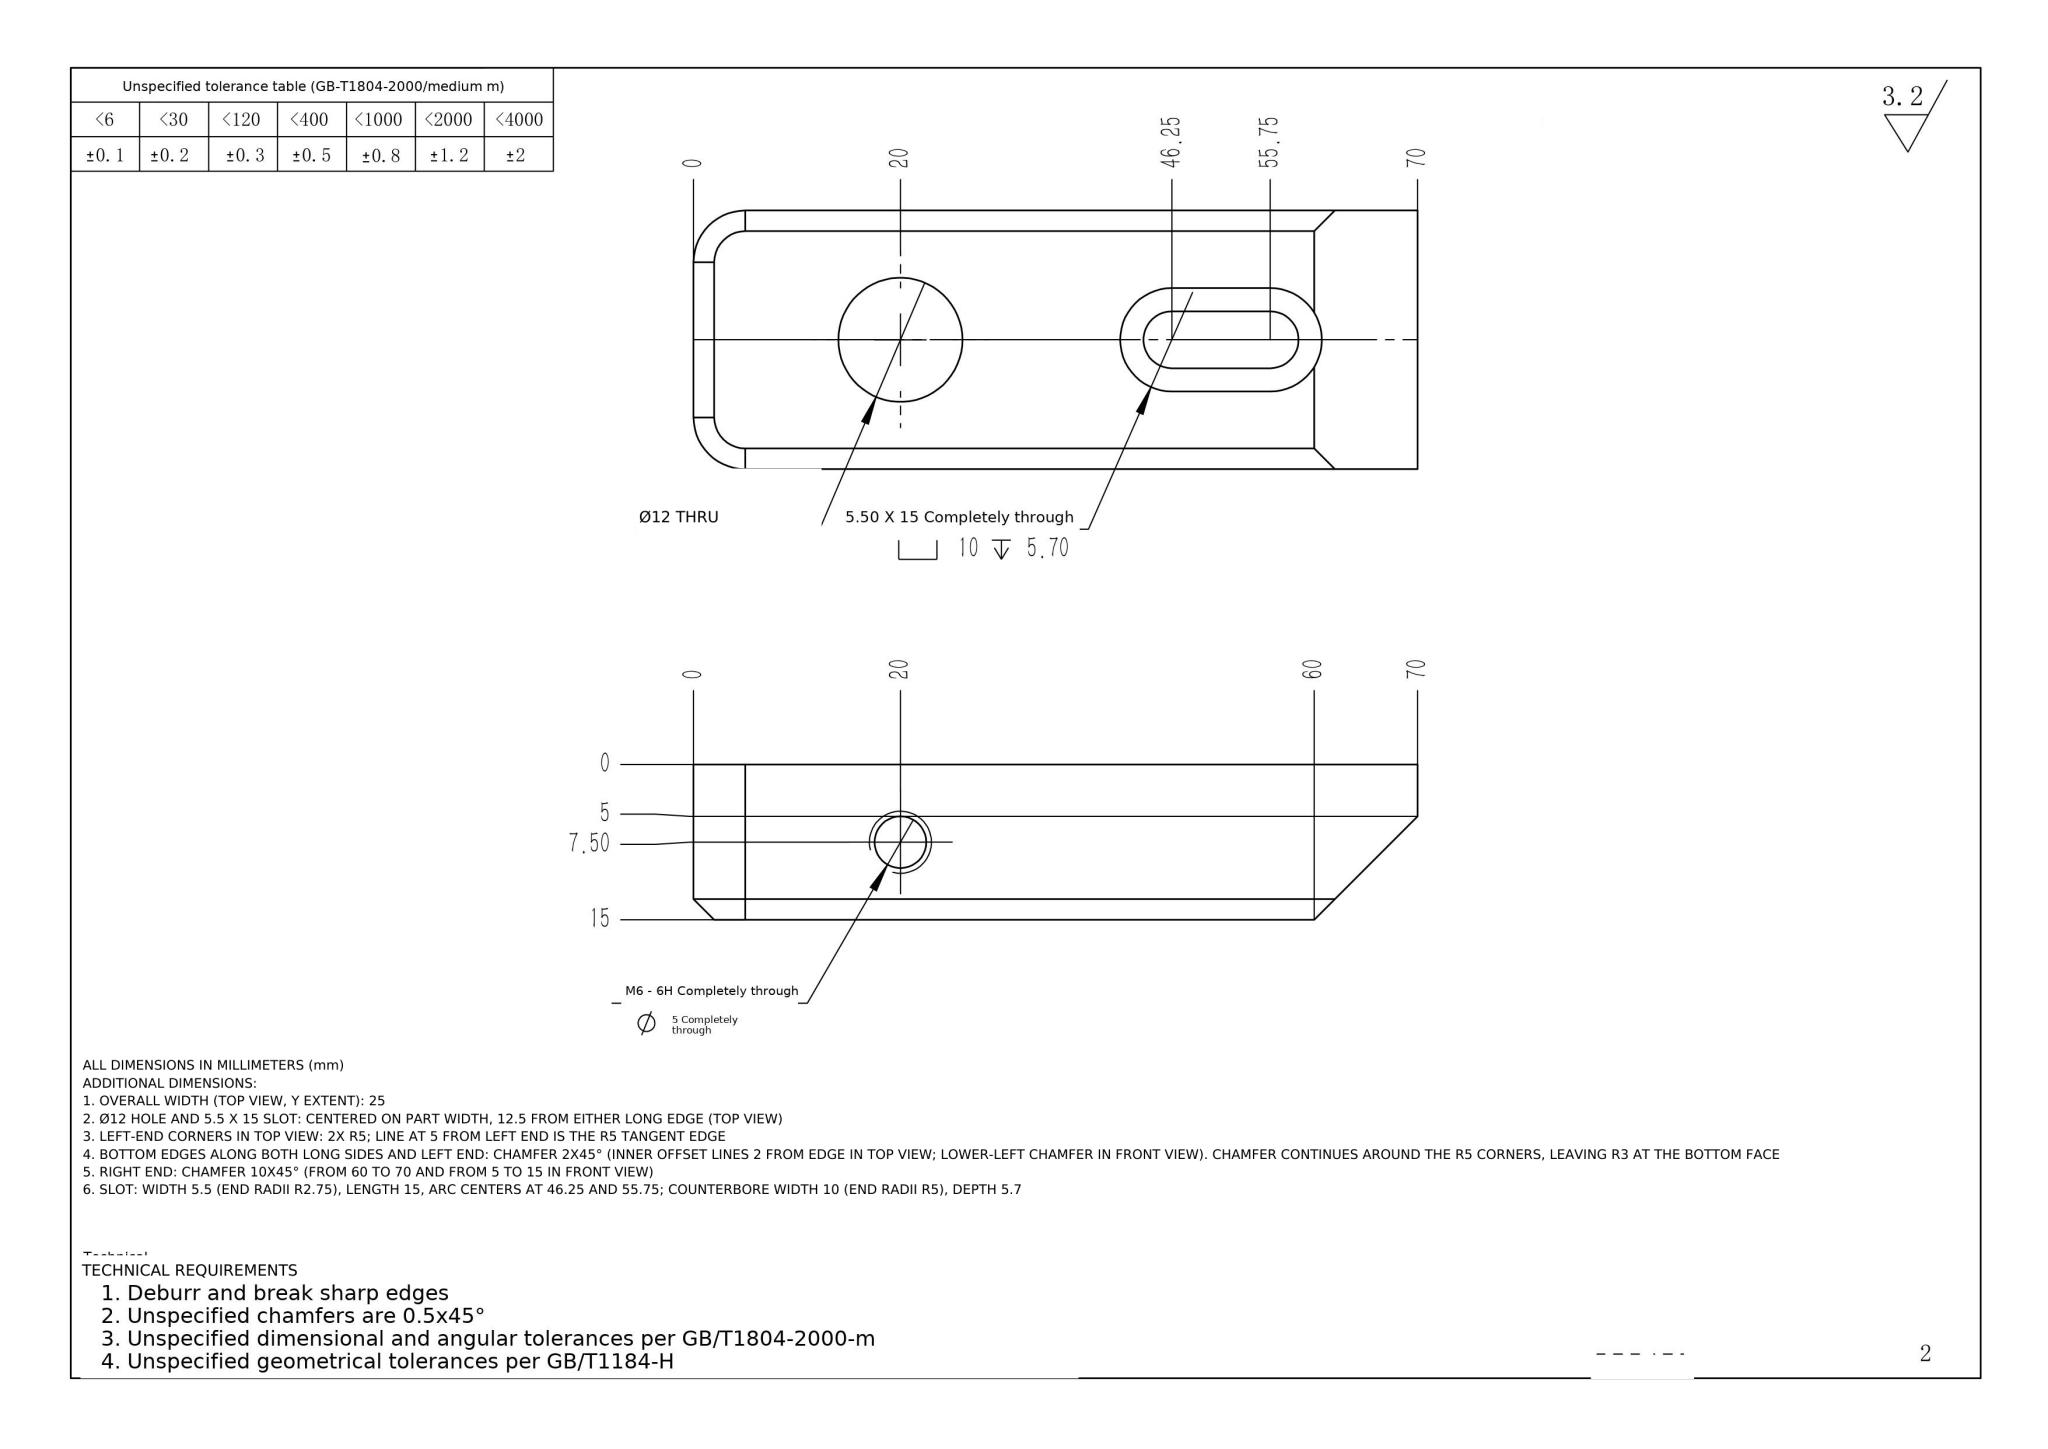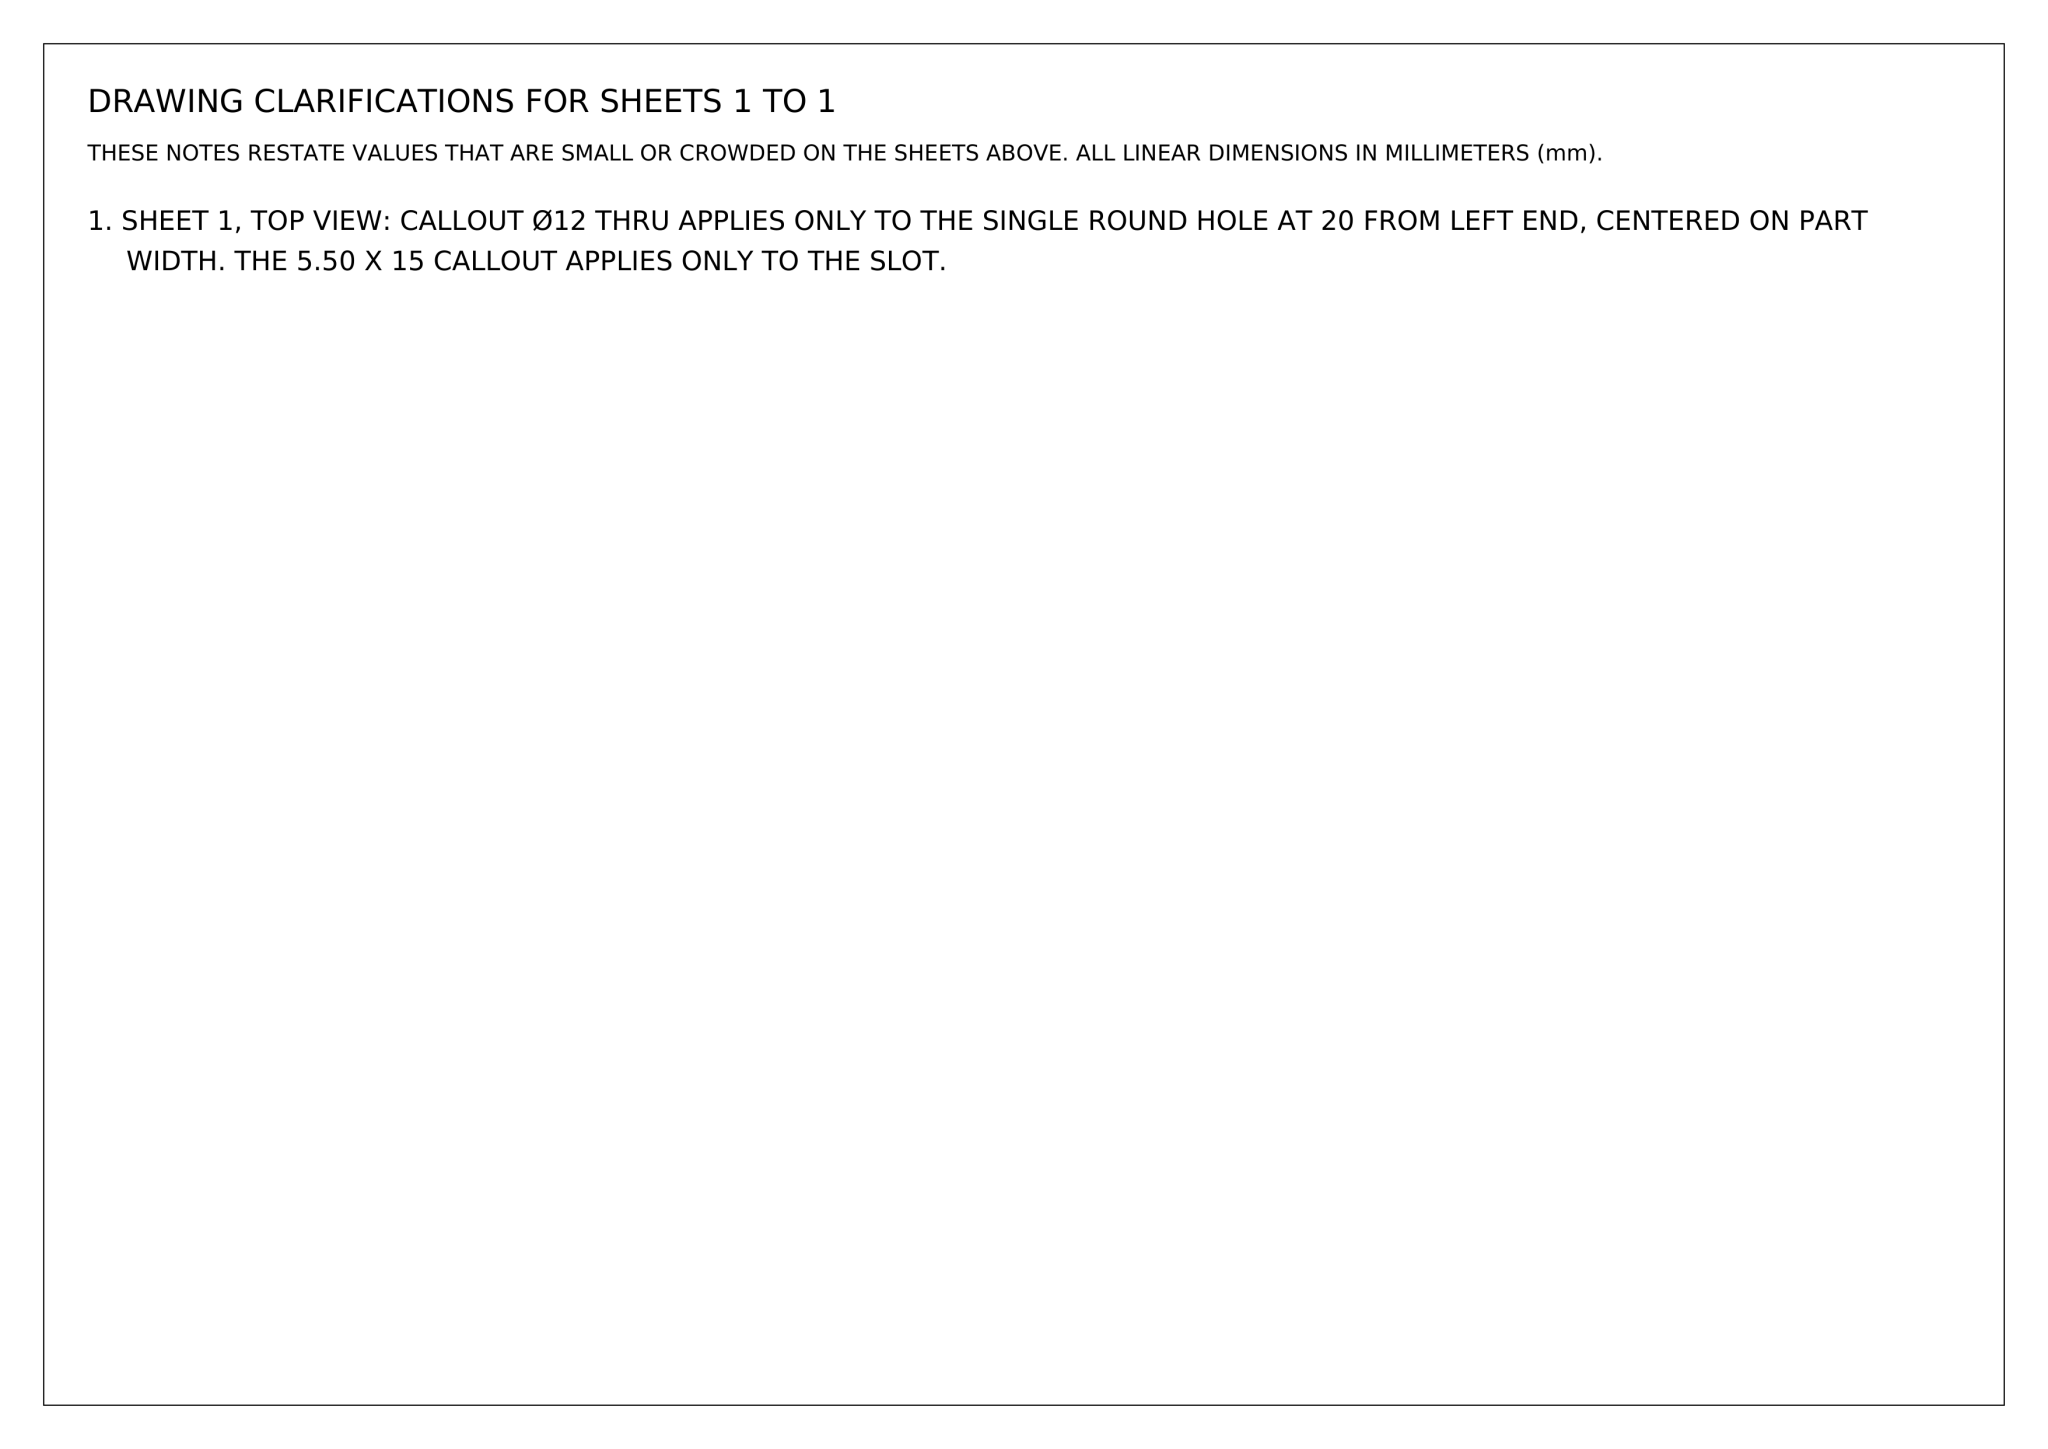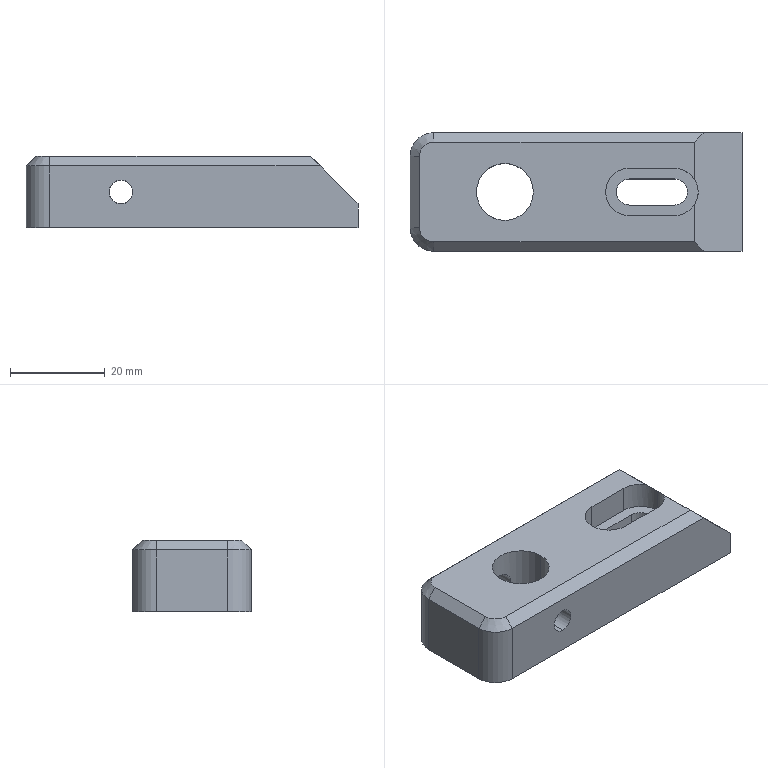Part | NX | mm | 1 solid | 31 faces | box 70 x 25 x 15 mm | volume 20907 mm3 | plane 15 | cylinder 14 | cone 2 | commonest cylinder face diameters 10 x5 5 x4 5.5 x3 12 x2